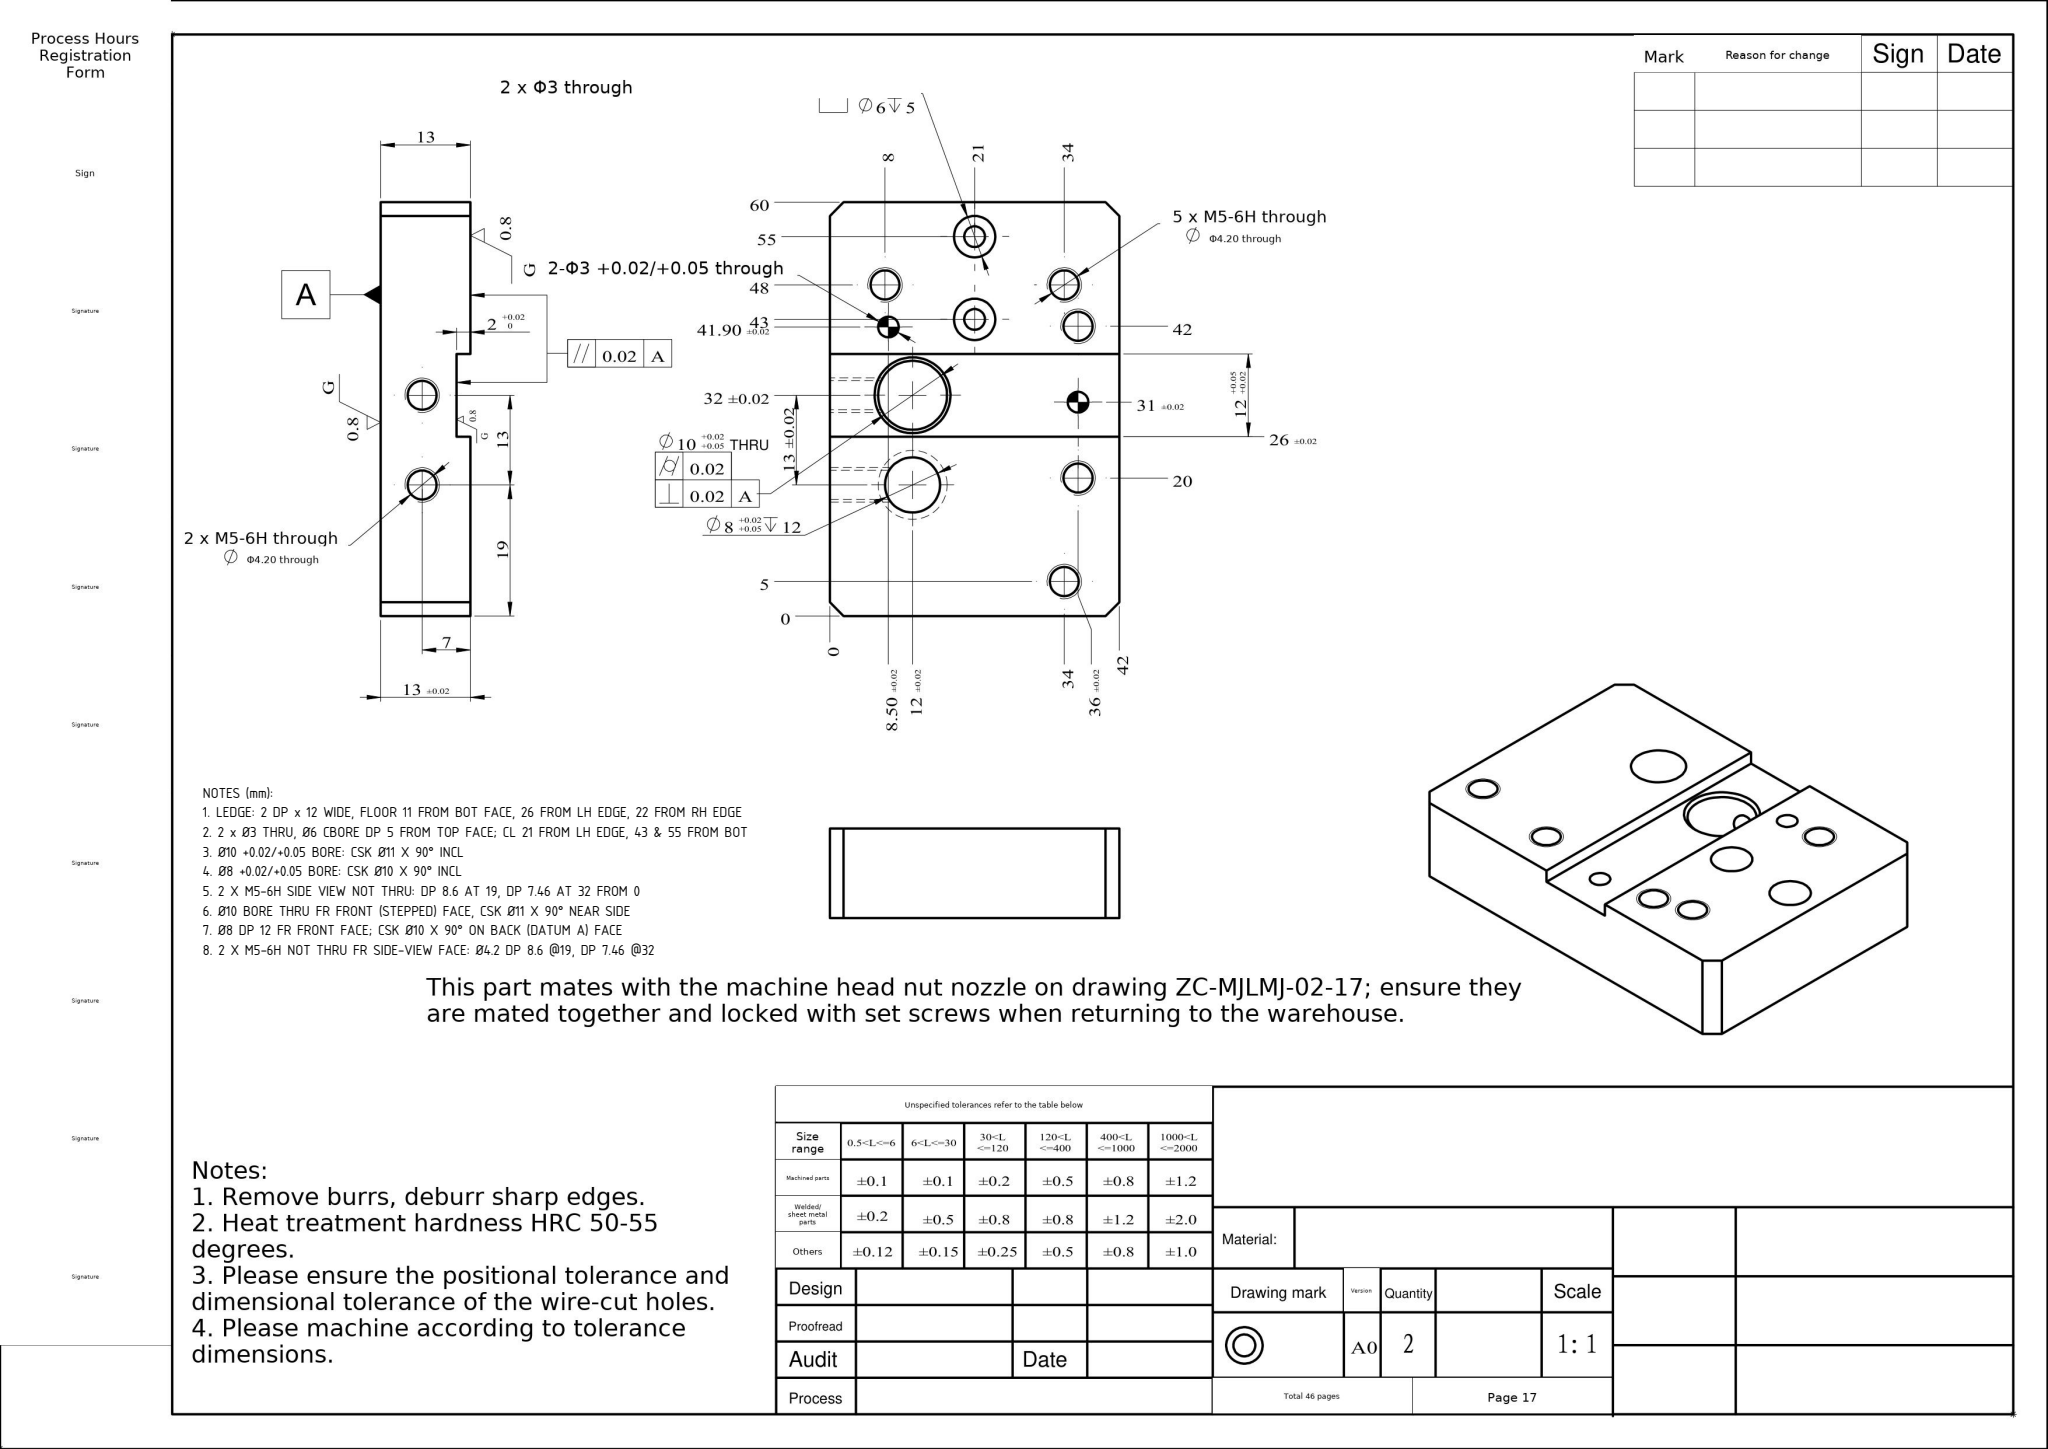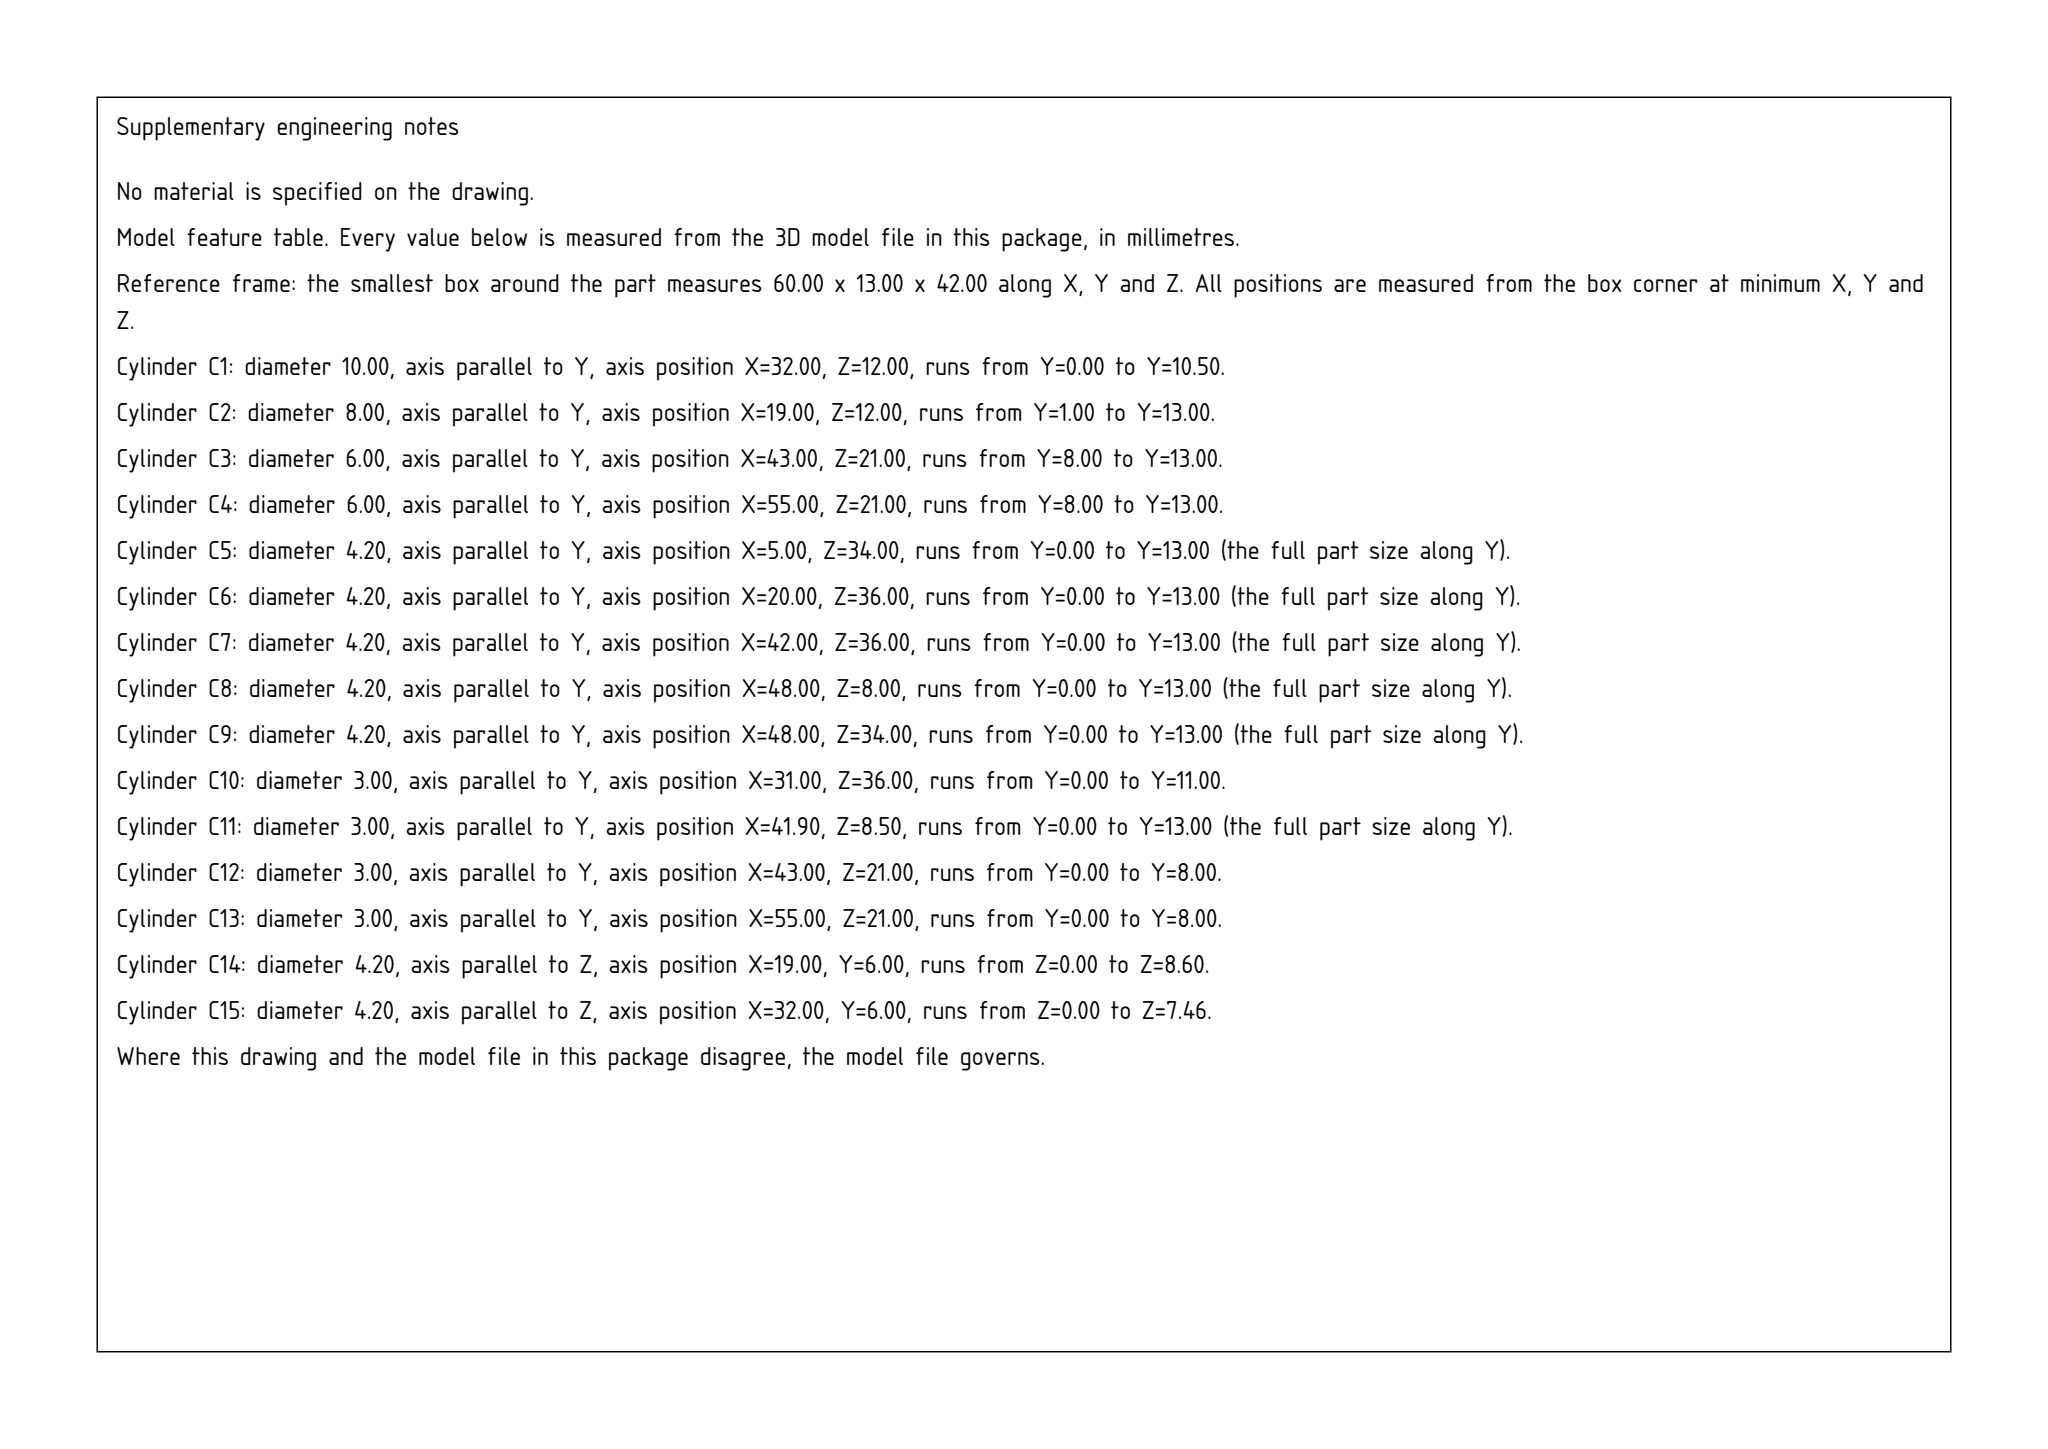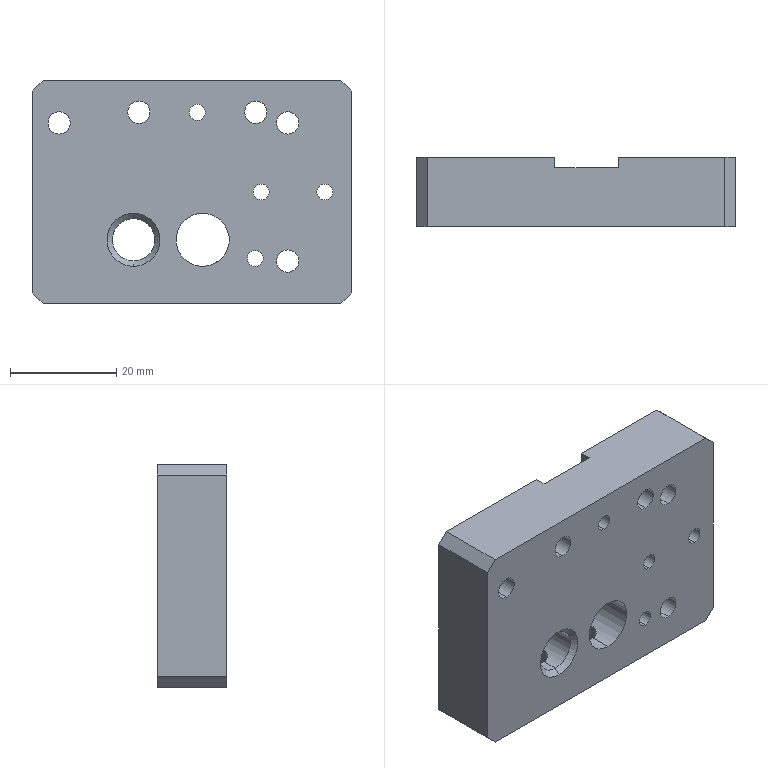Part | SolidWorks | mm | 1 solid | 50 faces | box 60 x 13 x 42 mm | volume 28436 mm3 | cylinder 30 | plane 16 | cone 4 | commonest cylinder face diameters 4.2 x14 3 x8 6 x4 8 x2 10 x2
Drawing notes:
LEDGE: 2 DP x 12 WIDE, FLOOR 11 FROM BOT FACE, 26 FROM LH EDGE, 22 FROM RH EDGE | from the solid: y-planes 0/11/13 (floor 2 below y=13); x-planes 26 & 38 bound 12-wide band, 60-38=22; Ø3 at x=31 len 11
2 x Ø3 THRU, Ø6 CBORE DP 5 FROM TOP FACE; CL 21 FROM LH EDGE, 43 & 55 FROM BOT | from the solid: Ø3 y-axis cyls at [43,21] & [55,21] len 8 + Ø6 same pos len 5, cbore floor y-plane 8.0; 8+5=13 thru
Ø10 +0.02/+0.05 BORE: CSK Ø11 X 90° INCL | from the solid: cones[90.0, ref_dia 11.0] coaxial with Ø10 y-axis bore at x32,z12
Ø8 +0.02/+0.05 BORE: CSK Ø10 X 90° INCL | from the solid: cones[90.0, ref_dia 10.0] coaxial with Ø8 y-axis bore at x19,z12
2 X M5-6H SIDE VIEW NOT THRU: DP 8.6 AT 19, DP 7.46 AT 32 FROM 0 | from the solid: cyl Ø4.2 axis z: (x19,y6) L=8.6 and (x32,y6) L=7.46, from z=0 face, breaking into Ø8/Ø10 bores
Ø10 BORE THRU FR FRONT (STEPPED) FACE, CSK Ø11 X 90° NEAR SIDE | from the solid: Ø10 y-axis cyl at x32,z12, L=10.5 in 11 thk step zone (y-planes 11 & 13); cone 90°, ref dia 11; 10.5+0.5=11 => breaks thru at y=11 step face
Ø8 DP 12 FR FRONT FACE; CSK Ø10 X 90° ON BACK (DATUM A) FACE | from the solid: Ø8 y-axis cyl at x19,z12, L=12 in 13 thk zone; cone 90° ref dia 10 => 1 deep; 12+1=13 full thk, csk on opposite face
2 X M5-6H NOT THRU FR SIDE-VIEW FACE: Ø4.2 DP 8.6 @19, DP 7.46 @32 | from the solid: Ø4.2 z-axis cyls at (x19,y6) L=8.6 and (x32,y6) L=7.46, part Z size 42 => blind
build123d program:
from build123d import *

# Parameters (mm, degrees)
SKETCH1_W              = 60
SKETCH1_H              = 42
BOSS_EXTRUDE1_DEPTH    = 13
CUT_EXTRUDE1_REACH     = 55.226
SKETCH2_W              = 12
SKETCH2_H              = 2
SKETCH3_R              = 5
SKETCH3_R_2            = 4
CUT_EXTRUDE2_DEPTH     = 13
M5_TAPPED_HOLE1_D      = 4.2
CUT_EXTRUDE4_REACH     = 40.859
SKETCH7_R              = 1.5
M5_TAPPED_HOLE2_REACH  = 55.226
M5_TAPPED_HOLE2_BORE_R = 2.1
CUT_EXTRUDE5_REACH     = 40.859
SKETCH10_R             = 1.5
SKETCH11_R             = 3
CUT_EXTRUDE6_DEPTH     = 5
CHAMFER2_SIZE          = 1
CHAMFER3_SIZE          = 0.5
CHAMFER4_SIZE          = 2


with BuildPart() as part:
    # Sketch1 → Boss-Extrude1 (new body)
    with BuildSketch(Plane(origin=(0, 0, 0), x_dir=(1, 0, 0), z_dir=(0, 1, 0))):
        Rectangle(SKETCH1_W, SKETCH1_H)
    extrude(amount=BOSS_EXTRUDE1_DEPTH)

    # Sketch2 → Cut-Extrude1 (cut, up to next)
    with BuildSketch(Plane.XY.offset(21), mode=Mode.PRIVATE) as cut_extrude1_sk1:
        with Locations((2, 12)):
            Rectangle(SKETCH2_W, SKETCH2_H)
    cut_extrude1_tool1 = extrude(cut_extrude1_sk1.sketch, amount=-CUT_EXTRUDE1_REACH, mode=Mode.PRIVATE) & part.part
    add(cut_extrude1_tool1.solids().sort_by_distance((2, 12, 21))[0], mode=Mode.SUBTRACT)

    # Sketch3 → Cut-Extrude2 (cut)
    with BuildSketch(Plane(origin=(0, 13, 0), x_dir=(1, 0, 0), z_dir=(0, 1, 0))):
        with Locations(Location((2, 9, 0), (0, 0, 270))):
            Circle(SKETCH3_R)
        with Locations(Location((-11, 9, 0), (0, 0, 270))):
            Circle(SKETCH3_R_2)
    extrude(amount=-CUT_EXTRUDE2_DEPTH, mode=Mode.SUBTRACT)

    # M5 Tapped Hole1 (through all)
    with Locations(Plane(origin=(0, 13, 0), x_dir=(1, 0, 0), z_dir=(0, 1, 0))):
        with Locations((18, 13), (18, -13), (-25, -13), (-10, -15), (12, -15)):
            Hole(M5_TAPPED_HOLE1_D / 2)

    # Sketch7 → Cut-Extrude4 (cut, up to next)
    with BuildSketch(Plane(origin=(0, 13, 0), x_dir=(1, 0, 0), z_dir=(0, 1, 0)), mode=Mode.PRIVATE) as cut_extrude4_sk1:
        with Locations(Location((1, -15, 0), (0, 0, 270))):
            Circle(SKETCH7_R)
    cut_extrude4_tool1 = extrude(cut_extrude4_sk1.sketch, amount=-CUT_EXTRUDE4_REACH, mode=Mode.PRIVATE) & part.part
    # Sketch7 → Cut-Extrude4 (cut, up to next)
    with BuildSketch(Plane(origin=(0, 13, 0), x_dir=(1, 0, 0), z_dir=(0, 1, 0)), mode=Mode.PRIVATE) as cut_extrude4_sk2:
        with Locations(Location((11.9, 12.5, 0), (0, 0, 270))):
            Circle(SKETCH7_R)
    cut_extrude4_tool2 = extrude(cut_extrude4_sk2.sketch, amount=-CUT_EXTRUDE4_REACH, mode=Mode.PRIVATE) & part.part
    add(cut_extrude4_tool1.solids().sort_by_distance((1, 13, 15))[0], mode=Mode.SUBTRACT)
    add(cut_extrude4_tool2.solids().sort_by_distance((11.9, 13, -12.5))[0], mode=Mode.SUBTRACT)

    # M5 Tapped Hole2 bore → M5 Tapped Hole2 (cut, up to next)
    with BuildSketch(Plane(origin=(0, 0, -21), x_dir=(-1, 0, 0), z_dir=(0, 0, -1)), mode=Mode.PRIVATE) as m5_tapped_hole2_sk1:
        with Locations((11, 6)):
            Circle(M5_TAPPED_HOLE2_BORE_R)
    m5_tapped_hole2_tool1 = extrude(m5_tapped_hole2_sk1.sketch, amount=-M5_TAPPED_HOLE2_REACH, mode=Mode.PRIVATE) & part.part
    # M5 Tapped Hole2 bore → M5 Tapped Hole2 (cut, up to next)
    with BuildSketch(Plane(origin=(0, 0, -21), x_dir=(-1, 0, 0), z_dir=(0, 0, -1)), mode=Mode.PRIVATE) as m5_tapped_hole2_sk2:
        with Locations((-2, 6)):
            Circle(M5_TAPPED_HOLE2_BORE_R)
    m5_tapped_hole2_tool2 = extrude(m5_tapped_hole2_sk2.sketch, amount=-M5_TAPPED_HOLE2_REACH, mode=Mode.PRIVATE) & part.part
    add(m5_tapped_hole2_tool1.solids().sort_by_distance((-11, 6, -21))[0], mode=Mode.SUBTRACT)
    add(m5_tapped_hole2_tool2.solids().sort_by_distance((2, 6, -21))[0], mode=Mode.SUBTRACT)

    # Sketch10 → Cut-Extrude5 (cut, up to next)
    with BuildSketch(Plane(origin=(0, 13, 0), x_dir=(1, 0, 0), z_dir=(0, 1, 0)), mode=Mode.PRIVATE) as cut_extrude5_sk1:
        with Locations(Location((25, 0, 0), (0, 0, 270))):
            Circle(SKETCH10_R)
    cut_extrude5_tool1 = extrude(cut_extrude5_sk1.sketch, amount=-CUT_EXTRUDE5_REACH, mode=Mode.PRIVATE) & part.part
    # Sketch10 → Cut-Extrude5 (cut, up to next)
    with BuildSketch(Plane(origin=(0, 13, 0), x_dir=(1, 0, 0), z_dir=(0, 1, 0)), mode=Mode.PRIVATE) as cut_extrude5_sk2:
        with Locations(Location((13, 0, 0), (0, 0, 270))):
            Circle(SKETCH10_R)
    cut_extrude5_tool2 = extrude(cut_extrude5_sk2.sketch, amount=-CUT_EXTRUDE5_REACH, mode=Mode.PRIVATE) & part.part
    add(cut_extrude5_tool1.solids().sort_by_distance((25, 13, 0))[0], mode=Mode.SUBTRACT)
    add(cut_extrude5_tool2.solids().sort_by_distance((13, 13, 0))[0], mode=Mode.SUBTRACT)

    # Sketch11 → Cut-Extrude6 (cut)
    with BuildSketch(Plane(origin=(0, 13, 0), x_dir=(1, 0, 0), z_dir=(0, 1, 0))):
        with Locations(Location((25, 0, 0), (0, 0, 270))):
            Circle(SKETCH11_R)
        with Locations(Location((13, 0, 0), (0, 0, 270))):
            Circle(SKETCH11_R)
    extrude(amount=-CUT_EXTRUDE6_DEPTH, mode=Mode.SUBTRACT)

    # Chamfer2
    chamfer2_edges = [part.edges().sort_by_distance(p)[0] for p in [
        (-11, 0, -13),
    ]]
    chamfer(chamfer2_edges, length=CHAMFER2_SIZE)

    # Chamfer3
    chamfer3_edges = [part.edges().sort_by_distance(p)[0] for p in [
        (2, 11, -14),
    ]]
    chamfer(chamfer3_edges, length=CHAMFER3_SIZE)

    # Chamfer4
    chamfer4_edges = [part.edges().sort_by_distance(p)[0] for p in [
        (30, 6.5, 21),
        (-30, 6.5, 21),
        (-30, 6.5, -21),
        (30, 6.5, -21),
    ]]
    chamfer(chamfer4_edges, length=CHAMFER4_SIZE)


solid = part.part